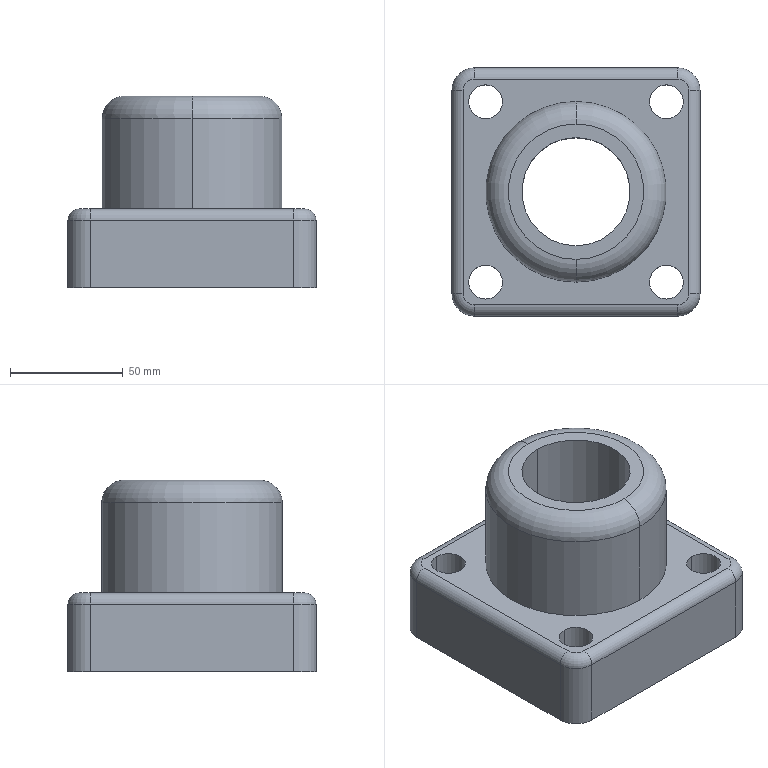Component | SolidWorks | CylinderJoint-1 | 1 solid | 36 faces | box 110 x 110 x 85 mm | volume 447298 mm3 | cylinder 22 | plane 8 | torus 6 | commonest cylinder face diameters 15 x8 10 x4 20 x4 48 x2 80 x2 85 x2 | material 1023 Carbon Steel Plate (SS)
STEP:
#1=CARTESIAN_POINT('',(-0.2935,1.047,21.063));
#2=VERTEX_POINT('',#1);
#3=CARTESIAN_POINT('',(-0.2935,-0.8432,21.063));
#4=VERTEX_POINT('',#3);
#5=CARTESIAN_POINT('',(-0.2935,0.1017,21.063));
#6=DIRECTION('',(-0.,-0.,-1.));
#7=DIRECTION('',(-0.,-1.,0.));
#8=AXIS2_PLACEMENT_3D('',#5,#6,#7);
#9=CIRCLE('',#8,0.9449);
#10=EDGE_CURVE('',#2,#4,#9,.T.);
#11=ORIENTED_EDGE('',*,*,#10,.T.);
#12=CARTESIAN_POINT('',(-0.2935,-0.8432,24.016));
#13=VERTEX_POINT('',#12);
#14=CARTESIAN_POINT('',(-0.2935,-0.8432,20.669));
#15=DIRECTION('',(0.,0.,1.));
#16=VECTOR('',#15,39.37);
#17=LINE('',#14,#16);
#18=EDGE_CURVE('',#4,#13,#17,.T.);
#19=ORIENTED_EDGE('',*,*,#18,.T.);
#20=CARTESIAN_POINT('',(-0.2935,1.047,24.016));
#21=VERTEX_POINT('',#20);
#22=CARTESIAN_POINT('',(-0.2935,0.1017,24.016));
#23=DIRECTION('',(0.,0.,1.));
#24=DIRECTION('',(0.,1.,0.));
#25=AXIS2_PLACEMENT_3D('',#22,#23,#24);
#26=CIRCLE('',#25,0.9449);
#27=EDGE_CURVE('',#13,#21,#26,.T.);
#28=ORIENTED_EDGE('',*,*,#27,.T.);
#29=CARTESIAN_POINT('',(-0.2935,1.047,20.669));
#30=DIRECTION('',(0.,0.,1.));
#31=VECTOR('',#30,39.37);
#32=LINE('',#29,#31);
#33=EDGE_CURVE('',#2,#21,#32,.T.);
#34=ORIENTED_EDGE('',*,*,#33,.F.);
#35=EDGE_LOOP('',(#11,#19,#28,#34));
#36=FACE_OUTER_BOUND('',#35,.T.);
#37=CARTESIAN_POINT('',(-0.2935,0.1017,20.669));
#38=DIRECTION('',(0.,0.,1.));
#39=DIRECTION('',(0.,1.,0.));
#40=AXIS2_PLACEMENT_3D('',#37,#38,#39);
#41=CYLINDRICAL_SURFACE('',#40,0.9449);
#42=ADVANCED_FACE('',(#36),#41,.F.);
#43=CARTESIAN_POINT('',(-0.2935,-1.473,23.622));
#44=VERTEX_POINT('',#43);
#45=CARTESIAN_POINT('',(-0.2935,1.677,23.622));
#46=VERTEX_POINT('',#45);
#47=CARTESIAN_POINT('',(-0.2935,0.1017,23.622));
#48=DIRECTION('',(-0.,-0.,-1.));
#49=DIRECTION('',(0.,1.,0.));
#50=AXIS2_PLACEMENT_3D('',#47,#48,#49);
#51=CIRCLE('',#50,1.575);
#52=EDGE_CURVE('',#44,#46,#51,.T.);
#53=ORIENTED_EDGE('',*,*,#52,.F.);
#54=CARTESIAN_POINT('',(-0.2935,-1.079,24.016));
#55=VERTEX_POINT('',#54);
#56=CARTESIAN_POINT('',(-0.2935,-1.079,23.622));
#57=DIRECTION('',(-1.,0.,0.));
#58=DIRECTION('',(-0.,-1.,0.));
#59=AXIS2_PLACEMENT_3D('',#56,#57,#58);
#60=CIRCLE('',#59,0.3937);
#61=EDGE_CURVE('',#44,#55,#60,.T.);
#62=ORIENTED_EDGE('',*,*,#61,.T.);
#63=CARTESIAN_POINT('',(-0.2935,1.283,24.016));
#64=VERTEX_POINT('',#63);
#65=CARTESIAN_POINT('',(-0.2935,0.1017,24.016));
#66=DIRECTION('',(0.,0.,1.));
#67=DIRECTION('',(0.,1.,0.));
#68=AXIS2_PLACEMENT_3D('',#65,#66,#67);
#69=CIRCLE('',#68,1.181);
#70=EDGE_CURVE('',#64,#55,#69,.T.);
#71=ORIENTED_EDGE('',*,*,#70,.F.);
#72=CARTESIAN_POINT('',(-0.2935,1.283,23.622));
#73=DIRECTION('',(1.,-0.,-0.));
#74=DIRECTION('',(0.,1.,0.));
#75=AXIS2_PLACEMENT_3D('',#72,#73,#74);
#76=CIRCLE('',#75,0.3937);
#77=EDGE_CURVE('',#46,#64,#76,.T.);
#78=ORIENTED_EDGE('',*,*,#77,.F.);
#79=EDGE_LOOP('',(#53,#62,#71,#78));
#80=FACE_OUTER_BOUND('',#79,.T.);
#81=CARTESIAN_POINT('',(-0.2935,0.1017,23.622));
#82=DIRECTION('',(0.,0.,1.));
#83=DIRECTION('',(0.,1.,-0.));
#84=AXIS2_PLACEMENT_3D('',#81,#82,#83);
#85=TOROIDAL_SURFACE('',#84,1.181,0.3937);
#86=ADVANCED_FACE('',(#80),#85,.T.);
#87=ORIENTED_EDGE('',*,*,#52,.T.);
#88=CARTESIAN_POINT('',(-0.2935,1.677,22.047));
#89=VERTEX_POINT('',#88);
#90=CARTESIAN_POINT('',(-0.2935,1.677,24.016));
#91=DIRECTION('',(-0.,-0.,-1.));
#92=VECTOR('',#91,39.37);
#93=LINE('',#90,#92);
#94=EDGE_CURVE('',#46,#89,#93,.T.);
#95=ORIENTED_EDGE('',*,*,#94,.T.);
#96=CARTESIAN_POINT('',(-0.2935,-1.473,22.047));
#97=VERTEX_POINT('',#96);
#98=CARTESIAN_POINT('',(-0.2935,0.1017,22.047));
#99=DIRECTION('',(0.,0.,1.));
#100=DIRECTION('',(0.,1.,0.));
#101=AXIS2_PLACEMENT_3D('',#98,#99,#100);
#102=CIRCLE('',#101,1.575);
#103=EDGE_CURVE('',#89,#97,#102,.T.);
#104=ORIENTED_EDGE('',*,*,#103,.T.);
#105=CARTESIAN_POINT('',(-0.2935,-1.473,24.016));
#106=DIRECTION('',(-0.,-0.,-1.));
#107=VECTOR('',#106,39.37);
#108=LINE('',#105,#107);
#109=EDGE_CURVE('',#44,#97,#108,.T.);
#110=ORIENTED_EDGE('',*,*,#109,.F.);
#111=EDGE_LOOP('',(#87,#95,#104,#110));
#112=FACE_OUTER_BOUND('',#111,.T.);
#113=CARTESIAN_POINT('',(-0.2935,0.1017,24.016));
#114=DIRECTION('',(-0.,-0.,-1.));
#115=DIRECTION('',(-0.,-1.,0.));
#116=AXIS2_PLACEMENT_3D('',#113,#114,#115);
#117=CYLINDRICAL_SURFACE('',#116,1.575);
#118=ADVANCED_FACE('',(#112),#117,.T.);
#119=CARTESIAN_POINT('',(1.281,-1.768,20.669));
#120=VERTEX_POINT('',#119);
#121=CARTESIAN_POINT('',(1.281,-1.178,20.669));
#122=VERTEX_POINT('',#121);
#123=CARTESIAN_POINT('',(1.281,-1.473,20.669));
#124=DIRECTION('',(0.,0.,1.));
#125=DIRECTION('',(0.,-1.,0.));
#126=AXIS2_PLACEMENT_3D('',#123,#124,#125);
#127=CIRCLE('',#126,0.2953);
#128=EDGE_CURVE('',#120,#122,#127,.T.);
#129=ORIENTED_EDGE('',*,*,#128,.F.);
#130=CARTESIAN_POINT('',(1.281,-1.768,22.047));
#131=VERTEX_POINT('',#130);
#132=CARTESIAN_POINT('',(1.281,-1.768,20.669));
#133=DIRECTION('',(0.,0.,1.));
#134=VECTOR('',#133,39.37);
#135=LINE('',#132,#134);
#136=EDGE_CURVE('',#120,#131,#135,.T.);
#137=ORIENTED_EDGE('',*,*,#136,.T.);
#138=CARTESIAN_POINT('',(1.281,-1.178,22.047));
#139=VERTEX_POINT('',#138);
#140=CARTESIAN_POINT('',(1.281,-1.473,22.047));
#141=DIRECTION('',(0.,0.,1.));
#142=DIRECTION('',(0.,-1.,0.));
#143=AXIS2_PLACEMENT_3D('',#140,#141,#142);
#144=CIRCLE('',#143,0.2953);
#145=EDGE_CURVE('',#131,#139,#144,.T.);
#146=ORIENTED_EDGE('',*,*,#145,.T.);
#147=CARTESIAN_POINT('',(1.281,-1.178,20.669));
#148=DIRECTION('',(0.,0.,1.));
#149=VECTOR('',#148,39.37);
#150=LINE('',#147,#149);
#151=EDGE_CURVE('',#122,#139,#150,.T.);
#152=ORIENTED_EDGE('',*,*,#151,.F.);
#153=EDGE_LOOP('',(#129,#137,#146,#152));
#154=FACE_OUTER_BOUND('',#153,.T.);
#155=CARTESIAN_POINT('',(1.281,-1.473,20.669));
#156=DIRECTION('',(0.,0.,1.));
#157=DIRECTION('',(0.,1.,0.));
#158=AXIS2_PLACEMENT_3D('',#155,#156,#157);
#159=CYLINDRICAL_SURFACE('',#158,0.2953);
#160=ADVANCED_FACE('',(#154),#159,.F.);
#161=CARTESIAN_POINT('',(1.281,1.381,20.669));
#162=VERTEX_POINT('',#161);
#163=CARTESIAN_POINT('',(1.281,1.972,20.669));
#164=VERTEX_POINT('',#163);
#165=CARTESIAN_POINT('',(1.281,1.677,20.669));
#166=DIRECTION('',(0.,0.,1.));
#167=DIRECTION('',(0.,1.,0.));
#168=AXIS2_PLACEMENT_3D('',#165,#166,#167);
#169=CIRCLE('',#168,0.2953);
#170=EDGE_CURVE('',#162,#164,#169,.T.);
#171=ORIENTED_EDGE('',*,*,#170,.F.);
#172=CARTESIAN_POINT('',(1.281,1.381,22.047));
#173=VERTEX_POINT('',#172);
#174=CARTESIAN_POINT('',(1.281,1.381,20.669));
#175=DIRECTION('',(0.,0.,1.));
#176=VECTOR('',#175,39.37);
#177=LINE('',#174,#176);
#178=EDGE_CURVE('',#162,#173,#177,.T.);
#179=ORIENTED_EDGE('',*,*,#178,.T.);
#180=CARTESIAN_POINT('',(1.281,1.972,22.047));
#181=VERTEX_POINT('',#180);
#182=CARTESIAN_POINT('',(1.281,1.677,22.047));
#183=DIRECTION('',(0.,0.,1.));
#184=DIRECTION('',(0.,1.,0.));
#185=AXIS2_PLACEMENT_3D('',#182,#183,#184);
#186=CIRCLE('',#185,0.2953);
#187=EDGE_CURVE('',#173,#181,#186,.T.);
#188=ORIENTED_EDGE('',*,*,#187,.T.);
#189=CARTESIAN_POINT('',(1.281,1.972,20.669));
#190=DIRECTION('',(0.,0.,1.));
#191=VECTOR('',#190,39.37);
#192=LINE('',#189,#191);
#193=EDGE_CURVE('',#164,#181,#192,.T.);
#194=ORIENTED_EDGE('',*,*,#193,.F.);
#195=EDGE_LOOP('',(#171,#179,#188,#194));
#196=FACE_OUTER_BOUND('',#195,.T.);
#197=CARTESIAN_POINT('',(1.281,1.677,20.669));
#198=DIRECTION('',(0.,0.,1.));
#199=DIRECTION('',(0.,1.,0.));
#200=AXIS2_PLACEMENT_3D('',#197,#198,#199);
#201=CYLINDRICAL_SURFACE('',#200,0.2953);
#202=ADVANCED_FACE('',(#196),#201,.F.);
#203=CARTESIAN_POINT('',(-1.868,1.381,20.669));
#204=VERTEX_POINT('',#203);
#205=CARTESIAN_POINT('',(-1.868,1.972,20.669));
#206=VERTEX_POINT('',#205);
#207=CARTESIAN_POINT('',(-1.868,1.677,20.669));
#208=DIRECTION('',(0.,0.,1.));
#209=DIRECTION('',(0.,-1.,0.));
#210=AXIS2_PLACEMENT_3D('',#207,#208,#209);
#211=CIRCLE('',#210,0.2953);
#212=EDGE_CURVE('',#204,#206,#211,.T.);
#213=ORIENTED_EDGE('',*,*,#212,.F.);
#214=CARTESIAN_POINT('',(-1.868,1.381,22.047));
#215=VERTEX_POINT('',#214);
#216=CARTESIAN_POINT('',(-1.868,1.381,20.669));
#217=DIRECTION('',(0.,0.,1.));
#218=VECTOR('',#217,39.37);
#219=LINE('',#216,#218);
#220=EDGE_CURVE('',#204,#215,#219,.T.);
#221=ORIENTED_EDGE('',*,*,#220,.T.);
#222=CARTESIAN_POINT('',(-1.868,1.972,22.047));
#223=VERTEX_POINT('',#222);
#224=CARTESIAN_POINT('',(-1.868,1.677,22.047));
#225=DIRECTION('',(0.,0.,1.));
#226=DIRECTION('',(0.,-1.,0.));
#227=AXIS2_PLACEMENT_3D('',#224,#225,#226);
#228=CIRCLE('',#227,0.2953);
#229=EDGE_CURVE('',#215,#223,#228,.T.);
#230=ORIENTED_EDGE('',*,*,#229,.T.);
#231=CARTESIAN_POINT('',(-1.868,1.972,20.669));
#232=DIRECTION('',(0.,0.,1.));
#233=VECTOR('',#232,39.37);
#234=LINE('',#231,#233);
#235=EDGE_CURVE('',#206,#223,#234,.T.);
#236=ORIENTED_EDGE('',*,*,#235,.F.);
#237=EDGE_LOOP('',(#213,#221,#230,#236));
#238=FACE_OUTER_BOUND('',#237,.T.);
#239=CARTESIAN_POINT('',(-1.868,1.677,20.669));
#240=DIRECTION('',(0.,0.,1.));
#241=DIRECTION('',(0.,1.,0.));
#242=AXIS2_PLACEMENT_3D('',#239,#240,#241);
#243=CYLINDRICAL_SURFACE('',#242,0.2953);
#244=ADVANCED_FACE('',(#238),#243,.F.);
#245=CARTESIAN_POINT('',(-1.868,-1.768,20.669));
#246=VERTEX_POINT('',#245);
#247=CARTESIAN_POINT('',(-1.868,-1.178,20.669));
#248=VERTEX_POINT('',#247);
#249=CARTESIAN_POINT('',(-1.868,-1.473,20.669));
#250=DIRECTION('',(0.,0.,1.));
#251=DIRECTION('',(0.,1.,0.));
#252=AXIS2_PLACEMENT_3D('',#249,#250,#251);
#253=CIRCLE('',#252,0.2953);
#254=EDGE_CURVE('',#246,#248,#253,.T.);
#255=ORIENTED_EDGE('',*,*,#254,.F.);
#256=CARTESIAN_POINT('',(-1.868,-1.768,22.047));
#257=VERTEX_POINT('',#256);
#258=CARTESIAN_POINT('',(-1.868,-1.768,20.669));
#259=DIRECTION('',(0.,0.,1.));
#260=VECTOR('',#259,39.37);
#261=LINE('',#258,#260);
#262=EDGE_CURVE('',#246,#257,#261,.T.);
#263=ORIENTED_EDGE('',*,*,#262,.T.);
#264=CARTESIAN_POINT('',(-1.868,-1.178,22.047));
#265=VERTEX_POINT('',#264);
#266=CARTESIAN_POINT('',(-1.868,-1.473,22.047));
#267=DIRECTION('',(0.,0.,1.));
#268=DIRECTION('',(0.,1.,0.));
#269=AXIS2_PLACEMENT_3D('',#266,#267,#268);
#270=CIRCLE('',#269,0.2953);
#271=EDGE_CURVE('',#257,#265,#270,.T.);
#272=ORIENTED_EDGE('',*,*,#271,.T.);
#273=CARTESIAN_POINT('',(-1.868,-1.178,20.669));
#274=DIRECTION('',(0.,0.,1.));
#275=VECTOR('',#274,39.37);
#276=LINE('',#273,#275);
#277=EDGE_CURVE('',#248,#265,#276,.T.);
#278=ORIENTED_EDGE('',*,*,#277,.F.);
#279=EDGE_LOOP('',(#255,#263,#272,#278));
#280=FACE_OUTER_BOUND('',#279,.T.);
#281=CARTESIAN_POINT('',(-1.868,-1.473,20.669));
#282=DIRECTION('',(0.,0.,1.));
#283=DIRECTION('',(0.,1.,0.));
#284=AXIS2_PLACEMENT_3D('',#281,#282,#283);
#285=CYLINDRICAL_SURFACE('',#284,0.2953);
#286=ADVANCED_FACE('',(#280),#285,.F.);
#287=CARTESIAN_POINT('',(-0.2935,1.775,21.063));
#288=VERTEX_POINT('',#287);
#289=CARTESIAN_POINT('',(-0.2935,-1.572,21.063));
#290=VERTEX_POINT('',#289);
#291=CARTESIAN_POINT('',(-0.2935,0.1017,21.063));
#292=DIRECTION('',(-0.,-0.,-1.));
#293=DIRECTION('',(-0.,-1.,0.));
#294=AXIS2_PLACEMENT_3D('',#291,#292,#293);
#295=CIRCLE('',#294,1.673);
#296=EDGE_CURVE('',#288,#290,#295,.T.);
#297=ORIENTED_EDGE('',*,*,#296,.F.);
#298=CARTESIAN_POINT('',(-0.2935,1.775,20.669));
#299=VERTEX_POINT('',#298);
#300=CARTESIAN_POINT('',(-0.2935,1.775,21.063));
#301=DIRECTION('',(-0.,-0.,-1.));
#302=VECTOR('',#301,39.37);
#303=LINE('',#300,#302);
#304=EDGE_CURVE('',#288,#299,#303,.T.);
#305=ORIENTED_EDGE('',*,*,#304,.T.);
#306=CARTESIAN_POINT('',(-0.2935,-1.572,20.669));
#307=VERTEX_POINT('',#306);
#308=CARTESIAN_POINT('',(-0.2935,0.1017,20.669));
#309=DIRECTION('',(-0.,-0.,-1.));
#310=DIRECTION('',(-0.,-1.,0.));
#311=AXIS2_PLACEMENT_3D('',#308,#309,#310);
#312=CIRCLE('',#311,1.673);
#313=EDGE_CURVE('',#299,#307,#312,.T.);
#314=ORIENTED_EDGE('',*,*,#313,.T.);
#315=CARTESIAN_POINT('',(-0.2935,-1.572,21.063));
#316=DIRECTION('',(-0.,-0.,-1.));
#317=VECTOR('',#316,39.37);
#318=LINE('',#315,#317);
#319=EDGE_CURVE('',#290,#307,#318,.T.);
#320=ORIENTED_EDGE('',*,*,#319,.F.);
#321=EDGE_LOOP('',(#297,#305,#314,#320));
#322=FACE_OUTER_BOUND('',#321,.T.);
#323=CARTESIAN_POINT('',(-0.2935,0.1017,21.063));
#324=DIRECTION('',(-0.,-0.,-1.));
#325=DIRECTION('',(-0.,-1.,0.));
#326=AXIS2_PLACEMENT_3D('',#323,#324,#325);
#327=CYLINDRICAL_SURFACE('',#326,1.673);
#328=ADVANCED_FACE('',(#322),#327,.F.);
#329=CARTESIAN_POINT('',(-1.868,-1.473,22.047));
#330=DIRECTION('',(0.,0.,1.));
#331=DIRECTION('',(0.,1.,0.));
#332=AXIS2_PLACEMENT_3D('',#329,#330,#331);
#333=CIRCLE('',#332,0.2953);
#334=EDGE_CURVE('',#265,#257,#333,.T.);
#335=ORIENTED_EDGE('',*,*,#334,.F.);
#336=ORIENTED_EDGE('',*,*,#271,.F.);
#337=EDGE_LOOP('',(#335,#336));
#338=FACE_BOUND('',#337,.T.);
#339=CARTESIAN_POINT('',(-1.868,1.677,22.047));
#340=DIRECTION('',(0.,0.,1.));
#341=DIRECTION('',(0.,-1.,0.));
#342=AXIS2_PLACEMENT_3D('',#339,#340,#341);
#343=CIRCLE('',#342,0.2953);
#344=EDGE_CURVE('',#223,#215,#343,.T.);
#345=ORIENTED_EDGE('',*,*,#344,.F.);
#346=ORIENTED_EDGE('',*,*,#229,.F.);
#347=EDGE_LOOP('',(#345,#346));
#348=FACE_BOUND('',#347,.T.);
#349=CARTESIAN_POINT('',(1.281,1.677,22.047));
#350=DIRECTION('',(0.,0.,1.));
#351=DIRECTION('',(0.,1.,0.));
#352=AXIS2_PLACEMENT_3D('',#349,#350,#351);
#353=CIRCLE('',#352,0.2953);
#354=EDGE_CURVE('',#181,#173,#353,.T.);
#355=ORIENTED_EDGE('',*,*,#354,.F.);
#356=ORIENTED_EDGE('',*,*,#187,.F.);
#357=EDGE_LOOP('',(#355,#356));
#358=FACE_BOUND('',#357,.T.);
#359=CARTESIAN_POINT('',(1.281,-1.473,22.047));
#360=DIRECTION('',(0.,0.,1.));
#361=DIRECTION('',(0.,-1.,0.));
#362=AXIS2_PLACEMENT_3D('',#359,#360,#361);
#363=CIRCLE('',#362,0.2953);
#364=EDGE_CURVE('',#139,#131,#363,.T.);
#365=ORIENTED_EDGE('',*,*,#364,.F.);
#366=ORIENTED_EDGE('',*,*,#145,.F.);
#367=EDGE_LOOP('',(#365,#366));
#368=FACE_BOUND('',#367,.T.);
#369=CARTESIAN_POINT('',(-0.2935,0.1017,22.047));
#370=DIRECTION('',(0.,0.,1.));
#371=DIRECTION('',(0.,1.,0.));
#372=AXIS2_PLACEMENT_3D('',#369,#370,#371);
#373=CIRCLE('',#372,1.575);
#374=EDGE_CURVE('',#97,#89,#373,.T.);
#375=ORIENTED_EDGE('',*,*,#374,.F.);
#376=ORIENTED_EDGE('',*,*,#103,.F.);
#377=EDGE_LOOP('',(#375,#376));
#378=FACE_BOUND('',#377,.T.);
#379=CARTESIAN_POINT('',(1.478,2.07,22.047));
#380=VERTEX_POINT('',#379);
#381=CARTESIAN_POINT('',(1.675,1.873,22.047));
#382=VERTEX_POINT('',#381);
#383=CARTESIAN_POINT('',(1.478,1.873,22.047));
#384=DIRECTION('',(-0.,-0.,-1.));
#385=DIRECTION('',(0.,1.,0.));
#386=AXIS2_PLACEMENT_3D('',#383,#384,#385);
#387=CIRCLE('',#386,0.1969);
#388=EDGE_CURVE('',#380,#382,#387,.T.);
#389=ORIENTED_EDGE('',*,*,#388,.F.);
#390=CARTESIAN_POINT('',(-2.065,2.07,22.047));
#391=VERTEX_POINT('',#390);
#392=CARTESIAN_POINT('',(-2.459,2.07,22.047));
#393=DIRECTION('',(-1.,0.,0.));
#394=VECTOR('',#393,39.37);
#395=LINE('',#392,#394);
#396=EDGE_CURVE('',#380,#391,#395,.T.);
#397=ORIENTED_EDGE('',*,*,#396,.T.);
#398=CARTESIAN_POINT('',(-2.262,1.873,22.047));
#399=VERTEX_POINT('',#398);
#400=CARTESIAN_POINT('',(-2.065,1.873,22.047));
#401=DIRECTION('',(-0.,-0.,-1.));
#402=DIRECTION('',(0.,1.,0.));
#403=AXIS2_PLACEMENT_3D('',#400,#401,#402);
#404=CIRCLE('',#403,0.1969);
#405=EDGE_CURVE('',#399,#391,#404,.T.);
#406=ORIENTED_EDGE('',*,*,#405,.F.);
#407=CARTESIAN_POINT('',(-2.262,-1.67,22.047));
#408=VERTEX_POINT('',#407);
#409=CARTESIAN_POINT('',(-2.262,-2.064,22.047));
#410=DIRECTION('',(-0.,-1.,0.));
#411=VECTOR('',#410,39.37);
#412=LINE('',#409,#411);
#413=EDGE_CURVE('',#399,#408,#412,.T.);
#414=ORIENTED_EDGE('',*,*,#413,.T.);
#415=CARTESIAN_POINT('',(-2.065,-1.867,22.047));
#416=VERTEX_POINT('',#415);
#417=CARTESIAN_POINT('',(-2.065,-1.67,22.047));
#418=DIRECTION('',(-0.,-0.,-1.));
#419=DIRECTION('',(0.,1.,0.));
#420=AXIS2_PLACEMENT_3D('',#417,#418,#419);
#421=CIRCLE('',#420,0.1969);
#422=EDGE_CURVE('',#416,#408,#421,.T.);
#423=ORIENTED_EDGE('',*,*,#422,.F.);
#424=CARTESIAN_POINT('',(1.478,-1.867,22.047));
#425=VERTEX_POINT('',#424);
#426=CARTESIAN_POINT('',(1.872,-1.867,22.047));
#427=DIRECTION('',(1.,-0.,-0.));
#428=VECTOR('',#427,39.37);
#429=LINE('',#426,#428);
#430=EDGE_CURVE('',#416,#425,#429,.T.);
#431=ORIENTED_EDGE('',*,*,#430,.T.);
#432=CARTESIAN_POINT('',(1.675,-1.67,22.047));
#433=VERTEX_POINT('',#432);
#434=CARTESIAN_POINT('',(1.478,-1.67,22.047));
#435=DIRECTION('',(-0.,-0.,-1.));
#436=DIRECTION('',(0.,1.,0.));
#437=AXIS2_PLACEMENT_3D('',#434,#435,#436);
#438=CIRCLE('',#437,0.1969);
#439=EDGE_CURVE('',#433,#425,#438,.T.);
#440=ORIENTED_EDGE('',*,*,#439,.F.);
#441=CARTESIAN_POINT('',(1.675,2.267,22.047));
#442=DIRECTION('',(0.,1.,-0.));
#443=VECTOR('',#442,39.37);
#444=LINE('',#441,#443);
#445=EDGE_CURVE('',#433,#382,#444,.T.);
#446=ORIENTED_EDGE('',*,*,#445,.T.);
#447=EDGE_LOOP('',(#389,#397,#406,#414,#423,#431,#440,#446));
#448=FACE_OUTER_BOUND('',#447,.T.);
#449=CARTESIAN_POINT('',(-2.459,-2.064,22.047));
#450=DIRECTION('',(0.,0.,1.));
#451=DIRECTION('',(0.,1.,-0.));
#452=AXIS2_PLACEMENT_3D('',#449,#450,#451);
#453=PLANE('',#452);
#454=ADVANCED_FACE('',(#338,#348,#358,#368,#378,#448),#453,.T.);
#455=CARTESIAN_POINT('',(1.478,-2.064,21.85));
#456=VERTEX_POINT('',#455);
#457=CARTESIAN_POINT('',(-2.065,-2.064,21.85));
#458=VERTEX_POINT('',#457);
#459=CARTESIAN_POINT('',(-2.459,-2.064,21.85));
#460=DIRECTION('',(-1.,0.,0.));
#461=VECTOR('',#460,39.37);
#462=LINE('',#459,#461);
#463=EDGE_CURVE('',#456,#458,#462,.T.);
#464=ORIENTED_EDGE('',*,*,#463,.T.);
#465=CARTESIAN_POINT('',(-2.065,-2.064,20.669));
#466=VERTEX_POINT('',#465);
#467=CARTESIAN_POINT('',(-2.065,-2.064,22.047));
#468=DIRECTION('',(-0.,-0.,-1.));
#469=VECTOR('',#468,39.37);
#470=LINE('',#467,#469);
#471=EDGE_CURVE('',#458,#466,#470,.T.);
#472=ORIENTED_EDGE('',*,*,#471,.T.);
#473=CARTESIAN_POINT('',(1.478,-2.064,20.669));
#474=VERTEX_POINT('',#473);
#475=CARTESIAN_POINT('',(1.872,-2.064,20.669));
#476=DIRECTION('',(1.,-0.,-0.));
#477=VECTOR('',#476,39.37);
#478=LINE('',#475,#477);
#479=EDGE_CURVE('',#466,#474,#478,.T.);
#480=ORIENTED_EDGE('',*,*,#479,.T.);
#481=CARTESIAN_POINT('',(1.478,-2.064,22.047));
#482=DIRECTION('',(0.,0.,1.));
#483=VECTOR('',#482,39.37);
#484=LINE('',#481,#483);
#485=EDGE_CURVE('',#474,#456,#484,.T.);
#486=ORIENTED_EDGE('',*,*,#485,.T.);
#487=EDGE_LOOP('',(#464,#472,#480,#486));
#488=FACE_OUTER_BOUND('',#487,.T.);
#489=CARTESIAN_POINT('',(1.872,-2.064,22.047));
#490=DIRECTION('',(0.,1.,-0.));
#491=DIRECTION('',(-0.,-0.,-1.));
#492=AXIS2_PLACEMENT_3D('',#489,#490,#491);
#493=PLANE('',#492);
#494=ADVANCED_FACE('',(#488),#493,.F.);
#495=CARTESIAN_POINT('',(1.872,1.873,21.85));
#496=VERTEX_POINT('',#495);
#497=CARTESIAN_POINT('',(1.872,-1.67,21.85));
#498=VERTEX_POINT('',#497);
#499=CARTESIAN_POINT('',(1.872,-2.064,21.85));
#500=DIRECTION('',(-0.,-1.,0.));
#501=VECTOR('',#500,39.37);
#502=LINE('',#499,#501);
#503=EDGE_CURVE('',#496,#498,#502,.T.);
#504=ORIENTED_EDGE('',*,*,#503,.T.);
#505=CARTESIAN_POINT('',(1.872,-1.67,20.669));
#506=VERTEX_POINT('',#505);
#507=CARTESIAN_POINT('',(1.872,-1.67,22.047));
#508=DIRECTION('',(-0.,-0.,-1.));
#509=VECTOR('',#508,39.37);
#510=LINE('',#507,#509);
#511=EDGE_CURVE('',#498,#506,#510,.T.);
#512=ORIENTED_EDGE('',*,*,#511,.T.);
#513=CARTESIAN_POINT('',(1.872,1.873,20.669));
#514=VERTEX_POINT('',#513);
#515=CARTESIAN_POINT('',(1.872,2.267,20.669));
#516=DIRECTION('',(0.,1.,-0.));
#517=VECTOR('',#516,39.37);
#518=LINE('',#515,#517);
#519=EDGE_CURVE('',#506,#514,#518,.T.);
#520=ORIENTED_EDGE('',*,*,#519,.T.);
#521=CARTESIAN_POINT('',(1.872,1.873,22.047));
#522=DIRECTION('',(0.,0.,1.));
#523=VECTOR('',#522,39.37);
#524=LINE('',#521,#523);
#525=EDGE_CURVE('',#514,#496,#524,.T.);
#526=ORIENTED_EDGE('',*,*,#525,.T.);
#527=EDGE_LOOP('',(#504,#512,#520,#526));
#528=FACE_OUTER_BOUND('',#527,.T.);
#529=CARTESIAN_POINT('',(1.872,2.267,22.047));
#530=DIRECTION('',(-1.,0.,0.));
#531=DIRECTION('',(-0.,-1.,0.));
#532=AXIS2_PLACEMENT_3D('',#529,#530,#531);
#533=PLANE('',#532);
#534=ADVANCED_FACE('',(#528),#533,.F.);
#535=CARTESIAN_POINT('',(1.478,2.267,20.669));
#536=VERTEX_POINT('',#535);
#537=CARTESIAN_POINT('',(-2.065,2.267,20.669));
#538=VERTEX_POINT('',#537);
#539=CARTESIAN_POINT('',(1.872,2.267,20.669));
#540=DIRECTION('',(-1.,0.,0.));
#541=VECTOR('',#540,39.37);
#542=LINE('',#539,#541);
#543=EDGE_CURVE('',#536,#538,#542,.T.);
#544=ORIENTED_EDGE('',*,*,#543,.T.);
#545=CARTESIAN_POINT('',(-2.065,2.267,21.85));
#546=VERTEX_POINT('',#545);
#547=CARTESIAN_POINT('',(-2.065,2.267,22.047));
#548=DIRECTION('',(0.,0.,1.));
#549=VECTOR('',#548,39.37);
#550=LINE('',#547,#549);
#551=EDGE_CURVE('',#538,#546,#550,.T.);
#552=ORIENTED_EDGE('',*,*,#551,.T.);
#553=CARTESIAN_POINT('',(1.478,2.267,21.85));
#554=VERTEX_POINT('',#553);
#555=CARTESIAN_POINT('',(1.872,2.267,21.85));
#556=DIRECTION('',(1.,-0.,-0.));
#557=VECTOR('',#556,39.37);
#558=LINE('',#555,#557);
#559=EDGE_CURVE('',#546,#554,#558,.T.);
#560=ORIENTED_EDGE('',*,*,#559,.T.);
#561=CARTESIAN_POINT('',(1.478,2.267,22.047));
#562=DIRECTION('',(-0.,-0.,-1.));
#563=VECTOR('',#562,39.37);
#564=LINE('',#561,#563);
#565=EDGE_CURVE('',#554,#536,#564,.T.);
#566=ORIENTED_EDGE('',*,*,#565,.T.);
#567=EDGE_LOOP('',(#544,#552,#560,#566));
#568=FACE_OUTER_BOUND('',#567,.T.);
#569=CARTESIAN_POINT('',(1.872,2.267,22.047));
#570=DIRECTION('',(-0.,-1.,0.));
#571=DIRECTION('',(0.,0.,1.));
#572=AXIS2_PLACEMENT_3D('',#569,#570,#571);
#573=PLANE('',#572);
#574=ADVANCED_FACE('',(#568),#573,.F.);
#575=CARTESIAN_POINT('',(-2.459,1.873,20.669));
#576=VERTEX_POINT('',#575);
#577=CARTESIAN_POINT('',(-2.459,-1.67,20.669));
#578=VERTEX_POINT('',#577);
#579=CARTESIAN_POINT('',(-2.459,2.267,20.669));
#580=DIRECTION('',(-0.,-1.,0.));
#581=VECTOR('',#580,39.37);
#582=LINE('',#579,#581);
#583=EDGE_CURVE('',#576,#578,#582,.T.);
#584=ORIENTED_EDGE('',*,*,#583,.T.);
#585=CARTESIAN_POINT('',(-2.459,-1.67,21.85));
#586=VERTEX_POINT('',#585);
#587=CARTESIAN_POINT('',(-2.459,-1.67,22.047));
#588=DIRECTION('',(0.,0.,1.));
#589=VECTOR('',#588,39.37);
#590=LINE('',#587,#589);
#591=EDGE_CURVE('',#578,#586,#590,.T.);
#592=ORIENTED_EDGE('',*,*,#591,.T.);
#593=CARTESIAN_POINT('',(-2.459,1.873,21.85));
#594=VERTEX_POINT('',#593);
#595=CARTESIAN_POINT('',(-2.459,2.267,21.85));
#596=DIRECTION('',(0.,1.,-0.));
#597=VECTOR('',#596,39.37);
#598=LINE('',#595,#597);
#599=EDGE_CURVE('',#586,#594,#598,.T.);
#600=ORIENTED_EDGE('',*,*,#599,.T.);
#601=CARTESIAN_POINT('',(-2.459,1.873,22.047));
#602=DIRECTION('',(-0.,-0.,-1.));
#603=VECTOR('',#602,39.37);
#604=LINE('',#601,#603);
#605=EDGE_CURVE('',#594,#576,#604,.T.);
#606=ORIENTED_EDGE('',*,*,#605,.T.);
#607=EDGE_LOOP('',(#584,#592,#600,#606));
#608=FACE_OUTER_BOUND('',#607,.T.);
#609=CARTESIAN_POINT('',(-2.459,2.267,22.047));
#610=DIRECTION('',(1.,-0.,-0.));
#611=DIRECTION('',(0.,1.,-0.));
#612=AXIS2_PLACEMENT_3D('',#609,#610,#611);
#613=PLANE('',#612);
#614=ADVANCED_FACE('',(#608),#613,.F.);
#615=CARTESIAN_POINT('',(1.281,-1.473,20.669));
#616=DIRECTION('',(0.,0.,1.));
#617=DIRECTION('',(0.,-1.,0.));
#618=AXIS2_PLACEMENT_3D('',#615,#616,#617);
#619=CIRCLE('',#618,0.2953);
#620=EDGE_CURVE('',#122,#120,#619,.T.);
#621=ORIENTED_EDGE('',*,*,#620,.T.);
#622=ORIENTED_EDGE('',*,*,#128,.T.);
#623=EDGE_LOOP('',(#621,#622));
#624=FACE_BOUND('',#623,.T.);
#625=CARTESIAN_POINT('',(1.281,1.677,20.669));
#626=DIRECTION('',(0.,0.,1.));
#627=DIRECTION('',(0.,1.,0.));
#628=AXIS2_PLACEMENT_3D('',#625,#626,#627);
#629=CIRCLE('',#628,0.2953);
#630=EDGE_CURVE('',#164,#162,#629,.T.);
#631=ORIENTED_EDGE('',*,*,#630,.T.);
#632=ORIENTED_EDGE('',*,*,#170,.T.);
#633=EDGE_LOOP('',(#631,#632));
#634=FACE_BOUND('',#633,.T.);
#635=CARTESIAN_POINT('',(-1.868,1.677,20.669));
#636=DIRECTION('',(0.,0.,1.));
#637=DIRECTION('',(0.,-1.,0.));
#638=AXIS2_PLACEMENT_3D('',#635,#636,#637);
#639=CIRCLE('',#638,0.2953);
#640=EDGE_CURVE('',#206,#204,#639,.T.);
#641=ORIENTED_EDGE('',*,*,#640,.T.);
#642=ORIENTED_EDGE('',*,*,#212,.T.);
#643=EDGE_LOOP('',(#641,#642));
#644=FACE_BOUND('',#643,.T.);
#645=CARTESIAN_POINT('',(-1.868,-1.473,20.669));
#646=DIRECTION('',(0.,0.,1.));
#647=DIRECTION('',(0.,1.,0.));
#648=AXIS2_PLACEMENT_3D('',#645,#646,#647);
#649=CIRCLE('',#648,0.2953);
#650=EDGE_CURVE('',#248,#246,#649,.T.);
#651=ORIENTED_EDGE('',*,*,#650,.T.);
#652=ORIENTED_EDGE('',*,*,#254,.T.);
#653=EDGE_LOOP('',(#651,#652));
#654=FACE_BOUND('',#653,.T.);
#655=CARTESIAN_POINT('',(-0.2935,0.1017,20.669));
#656=DIRECTION('',(-0.,-0.,-1.));
#657=DIRECTION('',(-0.,-1.,0.));
#658=AXIS2_PLACEMENT_3D('',#655,#656,#657);
#659=CIRCLE('',#658,1.673);
#660=EDGE_CURVE('',#307,#299,#659,.T.);
#661=ORIENTED_EDGE('',*,*,#660,.F.);
#662=ORIENTED_EDGE('',*,*,#313,.F.);
#663=EDGE_LOOP('',(#661,#662));
#664=FACE_BOUND('',#663,.T.);
#665=ORIENTED_EDGE('',*,*,#479,.F.);
#666=CARTESIAN_POINT('',(-2.065,-1.67,20.669));
#667=DIRECTION('',(-0.,-0.,-1.));
#668=DIRECTION('',(0.,1.,0.));
#669=AXIS2_PLACEMENT_3D('',#666,#667,#668);
#670=CIRCLE('',#669,0.3937);
#671=EDGE_CURVE('',#466,#578,#670,.T.);
#672=ORIENTED_EDGE('',*,*,#671,.T.);
#673=ORIENTED_EDGE('',*,*,#583,.F.);
#674=CARTESIAN_POINT('',(-2.065,1.873,20.669));
#675=DIRECTION('',(-0.,-0.,-1.));
#676=DIRECTION('',(0.,1.,0.));
#677=AXIS2_PLACEMENT_3D('',#674,#675,#676);
#678=CIRCLE('',#677,0.3937);
#679=EDGE_CURVE('',#576,#538,#678,.T.);
#680=ORIENTED_EDGE('',*,*,#679,.T.);
#681=ORIENTED_EDGE('',*,*,#543,.F.);
#682=CARTESIAN_POINT('',(1.478,1.873,20.669));
#683=DIRECTION('',(-0.,-0.,-1.));
#684=DIRECTION('',(0.,1.,0.));
#685=AXIS2_PLACEMENT_3D('',#682,#683,#684);
#686=CIRCLE('',#685,0.3937);
#687=EDGE_CURVE('',#536,#514,#686,.T.);
#688=ORIENTED_EDGE('',*,*,#687,.T.);
#689=ORIENTED_EDGE('',*,*,#519,.F.);
#690=CARTESIAN_POINT('',(1.478,-1.67,20.669));
#691=DIRECTION('',(-0.,-0.,-1.));
#692=DIRECTION('',(-0.,1.,0.));
#693=AXIS2_PLACEMENT_3D('',#690,#691,#692);
#694=CIRCLE('',#693,0.3937);
#695=EDGE_CURVE('',#506,#474,#694,.T.);
#696=ORIENTED_EDGE('',*,*,#695,.T.);
#697=EDGE_LOOP('',(#665,#672,#673,#680,#681,#688,#689,#696));
#698=FACE_OUTER_BOUND('',#697,.T.);
#699=CARTESIAN_POINT('',(-2.459,-2.064,20.669));
#700=DIRECTION('',(0.,0.,1.));
#701=DIRECTION('',(0.,1.,-0.));
#702=AXIS2_PLACEMENT_3D('',#699,#700,#701);
#703=PLANE('',#702);
#704=ADVANCED_FACE('',(#624,#634,#644,#654,#664,#698),#703,.F.);
#705=ORIENTED_EDGE('',*,*,#304,.F.);
#706=CARTESIAN_POINT('',(-0.2935,0.1017,21.063));
#707=DIRECTION('',(-0.,-0.,-1.));
#708=DIRECTION('',(-0.,-1.,0.));
#709=AXIS2_PLACEMENT_3D('',#706,#707,#708);
#710=CIRCLE('',#709,1.673);
#711=EDGE_CURVE('',#290,#288,#710,.T.);
#712=ORIENTED_EDGE('',*,*,#711,.F.);
#713=ORIENTED_EDGE('',*,*,#319,.T.);
#714=ORIENTED_EDGE('',*,*,#660,.T.);
#715=EDGE_LOOP('',(#705,#712,#713,#714));
#716=FACE_OUTER_BOUND('',#715,.T.);
#717=CARTESIAN_POINT('',(-0.2935,0.1017,21.063));
#718=DIRECTION('',(-0.,-0.,-1.));
#719=DIRECTION('',(-0.,-1.,0.));
#720=AXIS2_PLACEMENT_3D('',#717,#718,#719);
#721=CYLINDRICAL_SURFACE('',#720,1.673);
#722=ADVANCED_FACE('',(#716),#721,.F.);
#723=ORIENTED_EDGE('',*,*,#10,.F.);
#724=CARTESIAN_POINT('',(-0.2935,0.1017,21.063));
#725=DIRECTION('',(-0.,-0.,-1.));
#726=DIRECTION('',(-0.,-1.,0.));
#727=AXIS2_PLACEMENT_3D('',#724,#725,#726);
#728=CIRCLE('',#727,0.9449);
#729=EDGE_CURVE('',#4,#2,#728,.T.);
#730=ORIENTED_EDGE('',*,*,#729,.F.);
#731=EDGE_LOOP('',(#723,#730));
#732=FACE_BOUND('',#731,.T.);
#733=ORIENTED_EDGE('',*,*,#711,.T.);
#734=ORIENTED_EDGE('',*,*,#296,.T.);
#735=EDGE_LOOP('',(#733,#734));
#736=FACE_OUTER_BOUND('',#735,.T.);
#737=CARTESIAN_POINT('',(-0.2935,0.1017,21.063));
#738=DIRECTION('',(-0.,-0.,-1.));
#739=DIRECTION('',(-0.,-1.,0.));
#740=AXIS2_PLACEMENT_3D('',#737,#738,#739);
#741=PLANE('',#740);
#742=ADVANCED_FACE('',(#732,#736),#741,.T.);
#743=ORIENTED_EDGE('',*,*,#262,.F.);
#744=ORIENTED_EDGE('',*,*,#650,.F.);
#745=ORIENTED_EDGE('',*,*,#277,.T.);
#746=ORIENTED_EDGE('',*,*,#334,.T.);
#747=EDGE_LOOP('',(#743,#744,#745,#746));
#748=FACE_OUTER_BOUND('',#747,.T.);
#749=CARTESIAN_POINT('',(-1.868,-1.473,20.669));
#750=DIRECTION('',(0.,0.,1.));
#751=DIRECTION('',(0.,1.,0.));
#752=AXIS2_PLACEMENT_3D('',#749,#750,#751);
#753=CYLINDRICAL_SURFACE('',#752,0.2953);
#754=ADVANCED_FACE('',(#748),#753,.F.);
#755=ORIENTED_EDGE('',*,*,#220,.F.);
#756=ORIENTED_EDGE('',*,*,#640,.F.);
#757=ORIENTED_EDGE('',*,*,#235,.T.);
#758=ORIENTED_EDGE('',*,*,#344,.T.);
#759=EDGE_LOOP('',(#755,#756,#757,#758));
#760=FACE_OUTER_BOUND('',#759,.T.);
#761=CARTESIAN_POINT('',(-1.868,1.677,20.669));
#762=DIRECTION('',(0.,0.,1.));
#763=DIRECTION('',(0.,1.,0.));
#764=AXIS2_PLACEMENT_3D('',#761,#762,#763);
#765=CYLINDRICAL_SURFACE('',#764,0.2953);
#766=ADVANCED_FACE('',(#760),#765,.F.);
#767=ORIENTED_EDGE('',*,*,#178,.F.);
#768=ORIENTED_EDGE('',*,*,#630,.F.);
#769=ORIENTED_EDGE('',*,*,#193,.T.);
#770=ORIENTED_EDGE('',*,*,#354,.T.);
#771=EDGE_LOOP('',(#767,#768,#769,#770));
#772=FACE_OUTER_BOUND('',#771,.T.);
#773=CARTESIAN_POINT('',(1.281,1.677,20.669));
#774=DIRECTION('',(0.,0.,1.));
#775=DIRECTION('',(0.,1.,0.));
#776=AXIS2_PLACEMENT_3D('',#773,#774,#775);
#777=CYLINDRICAL_SURFACE('',#776,0.2953);
#778=ADVANCED_FACE('',(#772),#777,.F.);
#779=ORIENTED_EDGE('',*,*,#136,.F.);
#780=ORIENTED_EDGE('',*,*,#620,.F.);
#781=ORIENTED_EDGE('',*,*,#151,.T.);
#782=ORIENTED_EDGE('',*,*,#364,.T.);
#783=EDGE_LOOP('',(#779,#780,#781,#782));
#784=FACE_OUTER_BOUND('',#783,.T.);
#785=CARTESIAN_POINT('',(1.281,-1.473,20.669));
#786=DIRECTION('',(0.,0.,1.));
#787=DIRECTION('',(0.,1.,0.));
#788=AXIS2_PLACEMENT_3D('',#785,#786,#787);
#789=CYLINDRICAL_SURFACE('',#788,0.2953);
#790=ADVANCED_FACE('',(#784),#789,.F.);
#791=ORIENTED_EDGE('',*,*,#94,.F.);
#792=CARTESIAN_POINT('',(-0.2935,0.1017,23.622));
#793=DIRECTION('',(-0.,-0.,-1.));
#794=DIRECTION('',(0.,1.,0.));
#795=AXIS2_PLACEMENT_3D('',#792,#793,#794);
#796=CIRCLE('',#795,1.575);
#797=EDGE_CURVE('',#46,#44,#796,.T.);
#798=ORIENTED_EDGE('',*,*,#797,.T.);
#799=ORIENTED_EDGE('',*,*,#109,.T.);
#800=ORIENTED_EDGE('',*,*,#374,.T.);
#801=EDGE_LOOP('',(#791,#798,#799,#800));
#802=FACE_OUTER_BOUND('',#801,.T.);
#803=CARTESIAN_POINT('',(-0.2935,0.1017,24.016));
#804=DIRECTION('',(-0.,-0.,-1.));
#805=DIRECTION('',(-0.,-1.,0.));
#806=AXIS2_PLACEMENT_3D('',#803,#804,#805);
#807=CYLINDRICAL_SURFACE('',#806,1.575);
#808=ADVANCED_FACE('',(#802),#807,.T.);
#809=CARTESIAN_POINT('',(-0.2935,0.1017,24.016));
#810=DIRECTION('',(0.,0.,1.));
#811=DIRECTION('',(0.,1.,0.));
#812=AXIS2_PLACEMENT_3D('',#809,#810,#811);
#813=CIRCLE('',#812,0.9449);
#814=EDGE_CURVE('',#21,#13,#813,.T.);
#815=ORIENTED_EDGE('',*,*,#814,.F.);
#816=ORIENTED_EDGE('',*,*,#27,.F.);
#817=EDGE_LOOP('',(#815,#816));
#818=FACE_BOUND('',#817,.T.);
#819=ORIENTED_EDGE('',*,*,#70,.T.);
#820=CARTESIAN_POINT('',(-0.2935,0.1017,24.016));
#821=DIRECTION('',(0.,0.,1.));
#822=DIRECTION('',(0.,1.,0.));
#823=AXIS2_PLACEMENT_3D('',#820,#821,#822);
#824=CIRCLE('',#823,1.181);
#825=EDGE_CURVE('',#55,#64,#824,.T.);
#826=ORIENTED_EDGE('',*,*,#825,.T.);
#827=EDGE_LOOP('',(#819,#826));
#828=FACE_OUTER_BOUND('',#827,.T.);
#829=CARTESIAN_POINT('',(-0.2935,0.1017,24.016));
#830=DIRECTION('',(0.,0.,1.));
#831=DIRECTION('',(0.,1.,-0.));
#832=AXIS2_PLACEMENT_3D('',#829,#830,#831);
#833=PLANE('',#832);
#834=ADVANCED_FACE('',(#818,#828),#833,.T.);
#835=ORIENTED_EDGE('',*,*,#503,.F.);
#836=CARTESIAN_POINT('',(1.675,1.873,21.85));
#837=DIRECTION('',(-0.,-1.,0.));
#838=DIRECTION('',(0.,0.,1.));
#839=AXIS2_PLACEMENT_3D('',#836,#837,#838);
#840=CIRCLE('',#839,0.1969);
#841=EDGE_CURVE('',#496,#382,#840,.T.);
#842=ORIENTED_EDGE('',*,*,#841,.T.);
#843=ORIENTED_EDGE('',*,*,#445,.F.);
#844=CARTESIAN_POINT('',(1.675,-1.67,21.85));
#845=DIRECTION('',(0.,1.,-0.));
#846=DIRECTION('',(0.,0.,-1.));
#847=AXIS2_PLACEMENT_3D('',#844,#845,#846);
#848=CIRCLE('',#847,0.1969);
#849=EDGE_CURVE('',#433,#498,#848,.T.);
#850=ORIENTED_EDGE('',*,*,#849,.T.);
#851=EDGE_LOOP('',(#835,#842,#843,#850));
#852=FACE_OUTER_BOUND('',#851,.T.);
#853=CARTESIAN_POINT('',(1.675,-2.064,21.85));
#854=DIRECTION('',(-0.,-1.,0.));
#855=DIRECTION('',(1.,0.,0.));
#856=AXIS2_PLACEMENT_3D('',#853,#854,#855);
#857=CYLINDRICAL_SURFACE('',#856,0.1969);
#858=ADVANCED_FACE('',(#852),#857,.T.);
#859=ORIENTED_EDGE('',*,*,#559,.F.);
#860=CARTESIAN_POINT('',(-2.065,2.07,21.85));
#861=DIRECTION('',(1.,-0.,-0.));
#862=DIRECTION('',(0.,0.,-1.));
#863=AXIS2_PLACEMENT_3D('',#860,#861,#862);
#864=CIRCLE('',#863,0.1969);
#865=EDGE_CURVE('',#546,#391,#864,.T.);
#866=ORIENTED_EDGE('',*,*,#865,.T.);
#867=ORIENTED_EDGE('',*,*,#396,.F.);
#868=CARTESIAN_POINT('',(1.478,2.07,21.85));
#869=DIRECTION('',(-1.,0.,0.));
#870=DIRECTION('',(0.,0.,1.));
#871=AXIS2_PLACEMENT_3D('',#868,#869,#870);
#872=CIRCLE('',#871,0.1969);
#873=EDGE_CURVE('',#380,#554,#872,.T.);
#874=ORIENTED_EDGE('',*,*,#873,.T.);
#875=EDGE_LOOP('',(#859,#866,#867,#874));
#876=FACE_OUTER_BOUND('',#875,.T.);
#877=CARTESIAN_POINT('',(-2.459,2.07,21.85));
#878=DIRECTION('',(1.,-0.,-0.));
#879=DIRECTION('',(0.,0.,-1.));
#880=AXIS2_PLACEMENT_3D('',#877,#878,#879);
#881=CYLINDRICAL_SURFACE('',#880,0.1969);
#882=ADVANCED_FACE('',(#876),#881,.T.);
#883=ORIENTED_EDGE('',*,*,#463,.F.);
#884=CARTESIAN_POINT('',(1.478,-1.867,21.85));
#885=DIRECTION('',(-1.,0.,0.));
#886=DIRECTION('',(0.,0.,1.));
#887=AXIS2_PLACEMENT_3D('',#884,#885,#886);
#888=CIRCLE('',#887,0.1969);
#889=EDGE_CURVE('',#456,#425,#888,.T.);
#890=ORIENTED_EDGE('',*,*,#889,.T.);
#891=ORIENTED_EDGE('',*,*,#430,.F.);
#892=CARTESIAN_POINT('',(-2.065,-1.867,21.85));
#893=DIRECTION('',(1.,-0.,-0.));
#894=DIRECTION('',(0.,0.,-1.));
#895=AXIS2_PLACEMENT_3D('',#892,#893,#894);
#896=CIRCLE('',#895,0.1969);
#897=EDGE_CURVE('',#416,#458,#896,.T.);
#898=ORIENTED_EDGE('',*,*,#897,.T.);
#899=EDGE_LOOP('',(#883,#890,#891,#898));
#900=FACE_OUTER_BOUND('',#899,.T.);
#901=CARTESIAN_POINT('',(-2.459,-1.867,21.85));
#902=DIRECTION('',(-1.,0.,0.));
#903=DIRECTION('',(0.,0.,1.));
#904=AXIS2_PLACEMENT_3D('',#901,#902,#903);
#905=CYLINDRICAL_SURFACE('',#904,0.1969);
#906=ADVANCED_FACE('',(#900),#905,.T.);
#907=ORIENTED_EDGE('',*,*,#599,.F.);
#908=CARTESIAN_POINT('',(-2.262,-1.67,21.85));
#909=DIRECTION('',(0.,1.,-0.));
#910=DIRECTION('',(0.,0.,-1.));
#911=AXIS2_PLACEMENT_3D('',#908,#909,#910);
#912=CIRCLE('',#911,0.1969);
#913=EDGE_CURVE('',#586,#408,#912,.T.);
#914=ORIENTED_EDGE('',*,*,#913,.T.);
#915=ORIENTED_EDGE('',*,*,#413,.F.);
#916=CARTESIAN_POINT('',(-2.262,1.873,21.85));
#917=DIRECTION('',(-0.,-1.,0.));
#918=DIRECTION('',(0.,0.,1.));
#919=AXIS2_PLACEMENT_3D('',#916,#917,#918);
#920=CIRCLE('',#919,0.1969);
#921=EDGE_CURVE('',#399,#594,#920,.T.);
#922=ORIENTED_EDGE('',*,*,#921,.T.);
#923=EDGE_LOOP('',(#907,#914,#915,#922));
#924=FACE_OUTER_BOUND('',#923,.T.);
#925=CARTESIAN_POINT('',(-2.262,-2.064,21.85));
#926=DIRECTION('',(0.,1.,-0.));
#927=DIRECTION('',(-1.,0.,0.));
#928=AXIS2_PLACEMENT_3D('',#925,#926,#927);
#929=CYLINDRICAL_SURFACE('',#928,0.1969);
#930=ADVANCED_FACE('',(#924),#929,.T.);
#931=ORIENTED_EDGE('',*,*,#61,.F.);
#932=ORIENTED_EDGE('',*,*,#797,.F.);
#933=ORIENTED_EDGE('',*,*,#77,.T.);
#934=ORIENTED_EDGE('',*,*,#825,.F.);
#935=EDGE_LOOP('',(#931,#932,#933,#934));
#936=FACE_OUTER_BOUND('',#935,.T.);
#937=CARTESIAN_POINT('',(-0.2935,0.1017,23.622));
#938=DIRECTION('',(0.,0.,1.));
#939=DIRECTION('',(0.,1.,-0.));
#940=AXIS2_PLACEMENT_3D('',#937,#938,#939);
#941=TOROIDAL_SURFACE('',#940,1.181,0.3937);
#942=ADVANCED_FACE('',(#936),#941,.T.);
#943=ORIENTED_EDGE('',*,*,#687,.F.);
#944=ORIENTED_EDGE('',*,*,#565,.F.);
#945=CARTESIAN_POINT('',(1.478,1.873,21.85));
#946=DIRECTION('',(0.,0.,1.));
#947=DIRECTION('',(0.,1.,0.));
#948=AXIS2_PLACEMENT_3D('',#945,#946,#947);
#949=CIRCLE('',#948,0.3937);
#950=EDGE_CURVE('',#496,#554,#949,.T.);
#951=ORIENTED_EDGE('',*,*,#950,.F.);
#952=ORIENTED_EDGE('',*,*,#525,.F.);
#953=EDGE_LOOP('',(#943,#944,#951,#952));
#954=FACE_OUTER_BOUND('',#953,.T.);
#955=CARTESIAN_POINT('',(1.478,1.873,22.047));
#956=DIRECTION('',(-0.,-0.,-1.));
#957=DIRECTION('',(0.,-1.,0.));
#958=AXIS2_PLACEMENT_3D('',#955,#956,#957);
#959=CYLINDRICAL_SURFACE('',#958,0.3937);
#960=ADVANCED_FACE('',(#954),#959,.T.);
#961=ORIENTED_EDGE('',*,*,#841,.F.);
#962=ORIENTED_EDGE('',*,*,#950,.T.);
#963=ORIENTED_EDGE('',*,*,#873,.F.);
#964=ORIENTED_EDGE('',*,*,#388,.T.);
#965=EDGE_LOOP('',(#961,#962,#963,#964));
#966=FACE_OUTER_BOUND('',#965,.T.);
#967=CARTESIAN_POINT('',(1.478,1.873,21.85));
#968=DIRECTION('',(0.,0.,1.));
#969=DIRECTION('',(-0.,1.,-0.));
#970=AXIS2_PLACEMENT_3D('',#967,#968,#969);
#971=TOROIDAL_SURFACE('',#970,0.1969,0.1969);
#972=ADVANCED_FACE('',(#966),#971,.T.);
#973=ORIENTED_EDGE('',*,*,#679,.F.);
#974=ORIENTED_EDGE('',*,*,#605,.F.);
#975=CARTESIAN_POINT('',(-2.065,1.873,21.85));
#976=DIRECTION('',(0.,0.,1.));
#977=DIRECTION('',(0.,1.,0.));
#978=AXIS2_PLACEMENT_3D('',#975,#976,#977);
#979=CIRCLE('',#978,0.3937);
#980=EDGE_CURVE('',#546,#594,#979,.T.);
#981=ORIENTED_EDGE('',*,*,#980,.F.);
#982=ORIENTED_EDGE('',*,*,#551,.F.);
#983=EDGE_LOOP('',(#973,#974,#981,#982));
#984=FACE_OUTER_BOUND('',#983,.T.);
#985=CARTESIAN_POINT('',(-2.065,1.873,22.047));
#986=DIRECTION('',(-0.,-0.,-1.));
#987=DIRECTION('',(0.,-1.,0.));
#988=AXIS2_PLACEMENT_3D('',#985,#986,#987);
#989=CYLINDRICAL_SURFACE('',#988,0.3937);
#990=ADVANCED_FACE('',(#984),#989,.T.);
#991=ORIENTED_EDGE('',*,*,#865,.F.);
#992=ORIENTED_EDGE('',*,*,#980,.T.);
#993=ORIENTED_EDGE('',*,*,#921,.F.);
#994=ORIENTED_EDGE('',*,*,#405,.T.);
#995=EDGE_LOOP('',(#991,#992,#993,#994));
#996=FACE_OUTER_BOUND('',#995,.T.);
#997=CARTESIAN_POINT('',(-2.065,1.873,21.85));
#998=DIRECTION('',(0.,0.,1.));
#999=DIRECTION('',(-0.,1.,-0.));
#1000=AXIS2_PLACEMENT_3D('',#997,#998,#999);
#1001=TOROIDAL_SURFACE('',#1000,0.1969,0.1969);
#1002=ADVANCED_FACE('',(#996),#1001,.T.);
#1003=ORIENTED_EDGE('',*,*,#695,.F.);
#1004=ORIENTED_EDGE('',*,*,#511,.F.);
#1005=CARTESIAN_POINT('',(1.478,-1.67,21.85));
#1006=DIRECTION('',(0.,0.,1.));
#1007=DIRECTION('',(0.,1.,0.));
#1008=AXIS2_PLACEMENT_3D('',#1005,#1006,#1007);
#1009=CIRCLE('',#1008,0.3937);
#1010=EDGE_CURVE('',#456,#498,#1009,.T.);
#1011=ORIENTED_EDGE('',*,*,#1010,.F.);
#1012=ORIENTED_EDGE('',*,*,#485,.F.);
#1013=EDGE_LOOP('',(#1003,#1004,#1011,#1012));
#1014=FACE_OUTER_BOUND('',#1013,.T.);
#1015=CARTESIAN_POINT('',(1.478,-1.67,22.047));
#1016=DIRECTION('',(-0.,-0.,-1.));
#1017=DIRECTION('',(0.,-1.,0.));
#1018=AXIS2_PLACEMENT_3D('',#1015,#1016,#1017);
#1019=CYLINDRICAL_SURFACE('',#1018,0.3937);
#1020=ADVANCED_FACE('',(#1014),#1019,.T.);
#1021=ORIENTED_EDGE('',*,*,#849,.F.);
#1022=ORIENTED_EDGE('',*,*,#439,.T.);
#1023=ORIENTED_EDGE('',*,*,#889,.F.);
#1024=ORIENTED_EDGE('',*,*,#1010,.T.);
#1025=EDGE_LOOP('',(#1021,#1022,#1023,#1024));
#1026=FACE_OUTER_BOUND('',#1025,.T.);
#1027=CARTESIAN_POINT('',(1.478,-1.67,21.85));
#1028=DIRECTION('',(0.,0.,1.));
#1029=DIRECTION('',(-0.,1.,-0.));
#1030=AXIS2_PLACEMENT_3D('',#1027,#1028,#1029);
#1031=TOROIDAL_SURFACE('',#1030,0.1969,0.1969);
#1032=ADVANCED_FACE('',(#1026),#1031,.T.);
#1033=ORIENTED_EDGE('',*,*,#671,.F.);
#1034=ORIENTED_EDGE('',*,*,#471,.F.);
#1035=CARTESIAN_POINT('',(-2.065,-1.67,21.85));
#1036=DIRECTION('',(0.,0.,1.));
#1037=DIRECTION('',(0.,1.,0.));
#1038=AXIS2_PLACEMENT_3D('',#1035,#1036,#1037);
#1039=CIRCLE('',#1038,0.3937);
#1040=EDGE_CURVE('',#586,#458,#1039,.T.);
#1041=ORIENTED_EDGE('',*,*,#1040,.F.);
#1042=ORIENTED_EDGE('',*,*,#591,.F.);
#1043=EDGE_LOOP('',(#1033,#1034,#1041,#1042));
#1044=FACE_OUTER_BOUND('',#1043,.T.);
#1045=CARTESIAN_POINT('',(-2.065,-1.67,22.047));
#1046=DIRECTION('',(-0.,-0.,-1.));
#1047=DIRECTION('',(0.,-1.,0.));
#1048=AXIS2_PLACEMENT_3D('',#1045,#1046,#1047);
#1049=CYLINDRICAL_SURFACE('',#1048,0.3937);
#1050=ADVANCED_FACE('',(#1044),#1049,.T.);
#1051=ORIENTED_EDGE('',*,*,#897,.F.);
#1052=ORIENTED_EDGE('',*,*,#422,.T.);
#1053=ORIENTED_EDGE('',*,*,#913,.F.);
#1054=ORIENTED_EDGE('',*,*,#1040,.T.);
#1055=EDGE_LOOP('',(#1051,#1052,#1053,#1054));
#1056=FACE_OUTER_BOUND('',#1055,.T.);
#1057=CARTESIAN_POINT('',(-2.065,-1.67,21.85));
#1058=DIRECTION('',(0.,0.,1.));
#1059=DIRECTION('',(-0.,1.,-0.));
#1060=AXIS2_PLACEMENT_3D('',#1057,#1058,#1059);
#1061=TOROIDAL_SURFACE('',#1060,0.1969,0.1969);
#1062=ADVANCED_FACE('',(#1056),#1061,.T.);
#1063=ORIENTED_EDGE('',*,*,#18,.F.);
#1064=ORIENTED_EDGE('',*,*,#729,.T.);
#1065=ORIENTED_EDGE('',*,*,#33,.T.);
#1066=ORIENTED_EDGE('',*,*,#814,.T.);
#1067=EDGE_LOOP('',(#1063,#1064,#1065,#1066));
#1068=FACE_OUTER_BOUND('',#1067,.T.);
#1069=CARTESIAN_POINT('',(-0.2935,0.1017,20.669));
#1070=DIRECTION('',(0.,0.,1.));
#1071=DIRECTION('',(0.,1.,0.));
#1072=AXIS2_PLACEMENT_3D('',#1069,#1070,#1071);
#1073=CYLINDRICAL_SURFACE('',#1072,0.9449);
#1074=ADVANCED_FACE('',(#1068),#1073,.F.);
#1075=CLOSED_SHELL('',(#42,#86,#118,#160,#202,#244,#286,#328,#454,#494,#534,#574,#614,#704,#722,#742,#754,#766,#778,#790,#808,#834,#858,#882,#906,#930,#942,#960,#972,#990,#1002,#1020,#1032,#1050,#1062,#1074));
#1076=MANIFOLD_SOLID_BREP('',#1075);
#1077=CARTESIAN_POINT('',(0.,0.,0.));
#1078=DIRECTION('',(0.,0.,1.));
#1079=DIRECTION('',(1.,0.,0.));
#1080=AXIS2_PLACEMENT_3D('',#1077,#1078,#1079);
#1081=(LENGTH_UNIT()NAMED_UNIT(*)SI_UNIT($,.METRE.));
#1082=LENGTH_MEASURE_WITH_UNIT(LENGTH_MEASURE(0.0254),#1081);
#1083=DIMENSIONAL_EXPONENTS(1.,0.,0.,0.,0.,0.,0.);
#1084=(CONVERSION_BASED_UNIT('',#1082)LENGTH_UNIT()NAMED_UNIT(#1083));
#1085=UNCERTAINTY_MEASURE_WITH_UNIT(LENGTH_MEASURE(0.00001),#1084,'','');
#1086=(NAMED_UNIT(*)PLANE_ANGLE_UNIT()SI_UNIT($,.RADIAN.));
#1087=(NAMED_UNIT(*)SI_UNIT($,.STERADIAN.)SOLID_ANGLE_UNIT());
#1088=(GEOMETRIC_REPRESENTATION_CONTEXT(3)GLOBAL_UNCERTAINTY_ASSIGNED_CONTEXT((#1085))GLOBAL_UNIT_ASSIGNED_CONTEXT((#1084,#1086,#1087))REPRESENTATION_CONTEXT('',''));
#1089=ADVANCED_BREP_SHAPE_REPRESENTATION('',(#1076,#1080),#1088);
#1090=COLOUR_RGB('',0.7922,0.8196,0.9333);
#1091=FILL_AREA_STYLE_COLOUR('',#1090);
#1092=FILL_AREA_STYLE('',(#1091));
#1093=SURFACE_STYLE_FILL_AREA(#1092);
#1094=SURFACE_SIDE_STYLE('',(#1093));
#1095=SURFACE_STYLE_USAGE(.BOTH.,#1094);
#1096=PRESENTATION_STYLE_ASSIGNMENT((#1095));
#1097=STYLED_ITEM('',(#1096),#1076);
#1098=PRESENTATION_LAYER_ASSIGNMENT('','',(#1097));
#1099=(LENGTH_UNIT()NAMED_UNIT(*)SI_UNIT($,.METRE.));
#1100=LENGTH_MEASURE_WITH_UNIT(LENGTH_MEASURE(0.0254),#1099);
#1101=DIMENSIONAL_EXPONENTS(1.,0.,0.,0.,0.,0.,0.);
#1102=(CONVERSION_BASED_UNIT('',#1100)LENGTH_UNIT()NAMED_UNIT(#1101));
#1103=UNCERTAINTY_MEASURE_WITH_UNIT(LENGTH_MEASURE(0.00001),#1102,'','');
#1104=(NAMED_UNIT(*)PLANE_ANGLE_UNIT()SI_UNIT($,.RADIAN.));
#1105=(NAMED_UNIT(*)SI_UNIT($,.STERADIAN.)SOLID_ANGLE_UNIT());
#1106=(GEOMETRIC_REPRESENTATION_CONTEXT(3)GLOBAL_UNCERTAINTY_ASSIGNED_CONTEXT((#1103))GLOBAL_UNIT_ASSIGNED_CONTEXT((#1102,#1104,#1105))REPRESENTATION_CONTEXT('',''));
#1107=MECHANICAL_DESIGN_GEOMETRIC_PRESENTATION_REPRESENTATION('',(#1097),#1106);